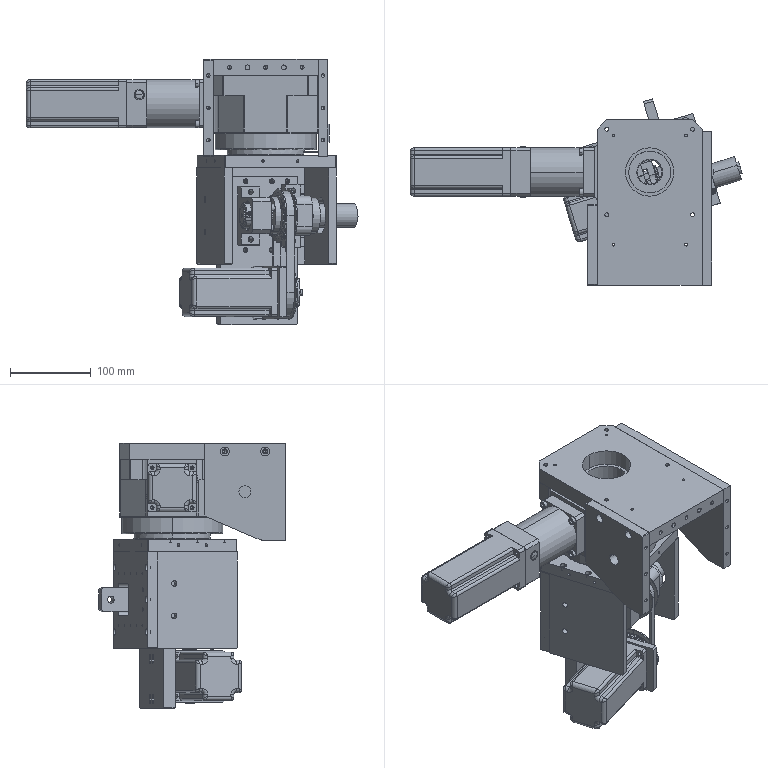Assembly | SolidWorks | mm | 53 component files | 55 solids | 3864 faces | box 411.09 x 231 x 328.5 mm | volume 4404841 mm3 | cylinder 1718 | plane 1389 | cone 489 | spline 222 | torus 46 | commonest cylinder face diameters 0.5 x176 0.4 x164 6.64 x156 5 x88 6 x86 52.53 x74 56.15 x72 3.3 x70
Bill of materials:
v1_Part1-2112091 | 1 |  | Thin-walled, closed band with an obround (stadium-shaped) outline: two straight parallel sides joined by semicircular ends, with a short constant axial width.
v1ZHXTbearingB6904ZZSB1 | 2 |  | Short annular body with a plain cylindrical bore, flat parallel faces, and concentric shallow recessed/stepped rings on the face. The overall look matches a sealed ball bearing.
V1ZHXTBearingMountingBaseSB1 | 1 |  | Block-style support with a large through-bore in a raised boss with chamfered corners, plus a thinner flange that sticks out on both sides and has one small through-hole in each tab. The overall look matches a shaft support or pillow-block bracket.
v1ZHXTRRING37SB1 | 1 |  | Thin flat split ring with two small lugs at the gap, each with a small round hole. The overall look matches a retaining ring (circlip).
V1ZHXTCylinderConnectionPlateSB1 | 1 |  | Rectangular block with chamfered corners, with one larger through-hole near one end and two smaller holes on an adjacent end face.
V1ZHXTGrindingBasePlateReinforcementPlateSB1 | 1 |  | Flat rectangular plate with two small through-holes near one edge on the main face and three small holes along one narrow edge face.
V1ZHXTGrindingBasePlateReinforcementRibSB1 | 1 |  | Flat rectangular plate with one large circular through-hole set off-center and three small holes along one narrow edge face.
v1ZHXTHG-KR23BSB1 | 1 |  | Simplified elongated rectangular housing with rounded edges and longitudinal recessed grooves on its sides. One end has a square flange with four corner holes, a circular pilot boss, and a protruding cylindrical shaft. The overall look matches a motor.
v1ZHXTHG-KR23SB1 | 1 |  | Elongated rectangular housing with rounded edges, longitudinal grooves, and a stepped/raised section at the rear end. The front has a square flange with four corner holes, a circular pilot, and a cylindrical shaft. The overall look matches a motor body.
v1ZHXTMGN12H--11SB1 | 2 |  | Long straight rail with a roughly rectangular cross-section, with longitudinal grooves along both sides near the top and a row of evenly spaced counterbored through-holes along its length. The overall look matches a linear guide rail.
v1ZHXTMGN12H-2SB1 | 4 |  | Rectangular carriage block with a channel underneath, with grooves inside the channel matching a rail profile. The flat top face has four holes in a rectangular pattern, and there are end plates/caps on both ends. The overall look matches a linear guide carriage.
V1ZHXTMotorMountingPlateSB1 | 1 |  | L-shaped bracket made from two plates at right angles. One plate has a large central circular opening with four small holes around it in a square pattern. The other leg has two mounting holes. Corners are chamfered.
v1ZHXTNKXRZ20SB1 | 1 |  | Stepped cylindrical sleeve or bushing with a through bore. The outer diameter has steps, and the outside has circumferential grooves. One end has a larger-diameter collar.
v1ZHXTHeadless_pin_DIN_913_M5x8SB1 | 3 |  | Short solid cylinder with a hexagonal socket recess in one end face and a chamfered or conical other end. The overall form looks like a set screw.
v1ZHXTPLNY20xSB1 | 1 |  | Annular ring with several rectangular slots evenly spaced around its outer edge and radial through-holes in the outer wall. The overall form looks like a slotted round nut or locking ring.
v1ZHXT14SB1 | 1 |  | Flanged hub: a circular flange with a central bore and a cylindrical, slightly tapered sleeve with a lengthwise slit on one side. Hex-socket cap-screw-like cylinders pass through the flange, and the flange also has plain holes.
v1ZHXTPTLA36P5M100_E_14_bodySB1 | 1 |  | Toothed pulley-like wheel with straight axial teeth and a raised disc flange on each side. It has a central bore and four small holes on a circle around the bore.
v1ZHXT20SB1 | 1 |  | Flanged hub similar to unnamed part 1: a circular flange with a central bore and a slit cylindrical sleeve on one side. Screw-like cylinders pass through the flange, and the flange also has plain holes.
v1ZHXTPTLA36P5M100_E_20_bodySB1 | 1 |  | Flanged toothed pulley-like wheel with straight axial teeth between two disc flanges and a central bore. Four small holes around the bore are visible from one face only.
V1ZHXTRotatingAxisMountingBaseSB1 | 1 |  | Bracket or support block: a flat mounting flange with two holes, joined to a body with rounded ends that holds a large cylindrical through bore. The bore axis is parallel to the mounting face.
V1ZHXTRotatingAxisSB1 | 1 |  | Stepped cylindrical shaft: a long, smaller-diameter section, a short intermediate step and a larger-diameter end section. The large end face has a small center hole, several small holes on a circle, and a circular step or groove.
V1ZHXTRotatingBasePlateSB1 | 1 |  | Thick rectangular plate with a large rectangular through cutout with rounded corners. It has rows of small holes, larger holes near the edges, and long shallow grooves across one face. One edge has a stepped or rebated strip.
V1ZHXTRotatingPlatformAdapterPlateSB1 | 1 | 6061 Alloy | Rectangular plate with a large central round through hole and many smaller holes in several sizes. The side edges also have holes.
V1ZHXTRotatingPlatformFixingPlateSB1 | 1 | 6061-O (SS) | Thick rectangular plate with two chamfered corners at one end, a large off-center round through hole, small holes in the face, and evenly spaced holes in the edge faces.
V1ZHXTRotatingSlideRailFixingPlateSB1 | 1 |  | Thin rectangular plate with many through holes: repeated groups of small holes in a grid, two clusters each with a larger central hole surrounded by smaller holes, and two pairs of short parallel slots toward one end.
V1ZHXT1,RR60BodySB1 | 1 |  | Housing-like body: a square flange with chamfered corners and four corner holes and a large central through bore, on top of a stepped cylindrical base; a cylindrical arm sticks out sideways and ends in a rectangular block with a small side hole.
V1ZHXT3.60InductionPlateSB1 | 1 |  | L-shaped bent bracket of thin sheet: a long flat leg with a rounded end and two through holes, and a short upright leg with a narrower stepped tab at the top.
v1ZHXTEE-SX672SB1 | 1 |  | Block-style bracket: an upright rectangular body with a slot cut into its bottom, forming two legs, and a horizontal cross-bar on top that extends into two rounded-end lugs, each with a through hole.
v1ZHXTHexagon socket button head screws GB_GB_SOCKET_TYPE7 M3X8-N_1SB1 | 4 |  | Pin with a plain cylindrical shank and a domed (round) head; looks like a rivet or round-head pin.
v1ZHXTHexagon socket countersunk head screws GB_GB_FASTENER_SCREWS_HSCHS M3X8-N_1SB1 | 8 |  | Pin with a cylindrical shank, a chamfered free end, and a conical head with a short cylindrical rim at its base; countersunk-head style.
v1ZHXTHexagon socket head cap screws GB_GB_FASTENER_SCREWS_HSHCS M5X20-N_1SB1 | 4 |  | Fastener-like pin: a cylindrical head with a rounded outer edge on a long cylindrical shank with a slightly chamfered end; resembles a socket-head cap screw envelope.
V1ZHXTZ-AxisConnectionPlateReinforcementRibSB1 | 1 |  | Thick flat plate with a mostly rectangular outline and one corner cut at an angle; it has a central through hole, two smaller holes near the top edge, and three small holes drilled into one narrow edge.
V1ZHXTZ-AxisMountingPlateReinforcementPlateSB1 | 1 |  | Tapered flat plate, like a gusset or bracket: tall at one end, sloping down along a straight angled edge toward the other end, with four evenly spaced holes along the long top edge and three small holes in the narrow edge at the tall end.
Mates:
1. concentric | V1ZHXTRotatingBasePlateSB1-1 face at (208.586, -137.891, 407.739) dir (-0.2918, 0.9565, 0) r 1.25 | v1ZHXTMGN12HSB1-1/v1ZHXTMGN12H--11SB1-1 face at (214.714, -157.977, 407.739) dir (0.2918, -0.9565, 0) r 1.75
2. concentric | V1ZHXTRotatingBasePlateSB1-1 face at (184.674, -145.187, 407.739) dir (-0.2918, 0.9565, 0) r 1.25 | v1ZHXTMGN12HSB1-1/v1ZHXTMGN12H--11SB1-1 face at (190.803, -165.272, 407.739) dir (0.2918, -0.9565, 0) r 1.75
3. concentric | V1ZHXTRotatingBasePlateSB1-1 face at (208.586, -137.891, 342.739) dir (-0.2918, 0.9565, 0) r 1.25 | v1ZHXTMGN12HSB1-2/v1ZHXTMGN12H--11SB1-1 face at (214.714, -157.977, 342.739) dir (0.2918, -0.9565, 0) r 1.75
4. concentric | V1ZHXTRotatingBasePlateSB1-1 face at (184.674, -145.187, 342.739) dir (-0.2918, 0.9565, 0) r 1.25 | v1ZHXTMGN12HSB1-2/v1ZHXTMGN12H--11SB1-1 face at (190.803, -165.272, 342.739) dir (0.2918, -0.9565, 0) r 1.75
5. coincident | V1ZHXTRotatingBasePlateSB1-1 face at (164.556, -164.917, 375.239) dir (0.2918, -0.9565, 0) | v1ZHXTMGN12HSB1-1/v1ZHXTMGN12H--11SB1-1 face at (164.556, -164.917, 407.739) dir (-0.2918, 0.9565, 0)
6. coincident | V1ZHXTRotatingBasePlateSB1-1 face at (164.556, -164.917, 375.239) dir (0.2918, -0.9565, 0) | v1ZHXTMGN12HSB1-2/v1ZHXTMGN12H--11SB1-1 face at (164.556, -164.917, 342.739) dir (-0.2918, 0.9565, 0)
7. coincident | v1ZHXTMGN12HSB1-2/v1ZHXTMGN12H-2SB1-3 face at (159.423, -180.074, 329.239) dir (0.2918, -0.9565, 0) | V1ZHXTRotatingSlideRailFixingPlateSB1-1 face at (163.536, -178.819, 375.239) dir (-0.2918, 0.9565, 0)
8. concentric | v1ZHXTMGN12HSB1-2/v1ZHXTMGN12H-2SB1-2 face at (198.926, -168.022, 332.739) dir (-0.2918, 0.9565, 0) r 1.5 | V1ZHXTRotatingSlideRailFixingPlateSB1-1 face at (203.303, -182.369, 332.739) dir (0.2918, -0.9565, 0) r 1.75
9. concentric | v1ZHXTMGN12HSB1-2/v1ZHXTMGN12H-2SB1-2 face at (198.926, -168.022, 352.739) dir (-0.2918, 0.9565, 0) r 1.5 | V1ZHXTRotatingSlideRailFixingPlateSB1-1 face at (203.303, -182.369, 352.739) dir (0.2918, -0.9565, 0) r 1.75
10. coincident | V1ZHXTRotatingSlideRailFixingPlateSB1-1 face at (167.914, -193.166, 375.239) dir (0.2918, -0.9565, 0) | V1ZHXTRotatingAxisMountingBaseSB1-1 face at (215.737, -178.575, 375.239) dir (-0.2918, 0.9565, 0)
11. concentric | V1ZHXTRotatingAxisMountingBaseSB1-1 face at (208.281, -222.67, 375.239) dir (0.9565, 0.2918, 0) r 18.5 | v1ZHXTNKXRZ20SB1-1 face at (209.238, -222.378, 375.239) dir (0.9565, 0.2918, 0) r 10
12. coincident | V1ZHXTRotatingAxisMountingBaseSB1-1 face at (234.123, -238.832, 336.239) dir (0.9565, 0.2918, 0) | v1ZHXTNKXRZ20SB1-1 face at (232.555, -233.696, 382.588) dir (-0.9565, -0.2918, 0)
13. concentric | V1ZHXTRotatingAxisSB1-1 face at (228.367, -216.542, 375.239) dir (-0.9565, -0.2918, 0) r 10 | v1ZHXTNKXRZ20SB1-1 face at (209.238, -222.378, 375.239) dir (0.9565, 0.2918, 0) r 10
14. coincident | V1ZHXTRotatingAxisSB1-1 face at (228.367, -216.542, 375.239) dir (-0.9565, -0.2918, 0) | v1ZHXTNKXRZ20SB1-1 face at (231.734, -227.577, 380.048) dir (0.9565, 0.2918, 0)
15. coincident | V1ZHXTRotatingSlideRailFixingPlateSB1-1 face at (167.914, -193.166, 375.239) dir (0.2918, -0.9565, 0) | V1ZHXTMotorMountingPlateSB1-1 face at (170.783, -192.291, 312.739) dir (-0.2918, 0.9565, 0)
16. coincident | V1ZHXTRotatingBasePlateSB1-1 face at (230.106, -131.325, 315.239) dir (0.9565, 0.2918, 0) | V1ZHXTRotatingPlatformAdapterPlateSB1-1 face at (223.394, -109.326, 435.239) dir (0.9565, 0.2918, 0)
17. coincident | V1ZHXTRotatingBasePlateSB1-1 face at (164.556, -164.917, 375.239) dir (0.2918, -0.9565, 0) | V1ZHXTGrindingBasePlateReinforcementPlateSB1-3 face at (104.777, -183.156, 435.239) dir (-0.2918, 0.9565, 0)
18. coincident | V1ZHXTRotatingPlatformAdapterPlateSB1-1 face at (230.106, -131.325, 435.239) dir (-0.2918, 0.9565, 0) | V1ZHXTRotatingBasePlateSB1-1 face at (160.762, -152.482, 375.239) dir (-0.2918, 0.9565, 0)
19. concentric | V1ZHXTRotatingSlideRailFixingPlateSB1-1 face at (170.232, -176.777, 255.239) dir (0.2918, -0.9565, 0) r 2.6 | V1ZHXTMotorMountingPlateSB1-1 face at (174.609, -191.124, 255.239) dir (-0.2918, 0.9565, 0) r 2.1
20. coincident | V1ZHXTRotatingSlideRailFixingPlateSB1-1 face at (167.914, -193.166, 375.239) dir (0.2918, -0.9565, 0) | v1ZHXTBGMWB6904ZZ_40SB1-1/V1ZHXTBearingMountingBaseSB1-1 face at (142.089, -201.046, 411.739) dir (-0.2918, 0.9565, 0)
21. concentric | V1ZHXTRotatingSlideRailFixingPlateSB1-1 face at (206.172, -181.493, 344.239) dir (0.2918, -0.9565, 0) r 2.5 | V1ZHXTRotatingAxisMountingBaseSB1-1 face at (206.172, -181.493, 344.239) dir (0.2918, -0.9565, 0) r 3.25
22. concentric | V1ZHXTRotatingSlideRailFixingPlateSB1-1 face at (206.172, -181.493, 406.239) dir (0.2918, -0.9565, 0) r 2.5 | V1ZHXTRotatingAxisMountingBaseSB1-1 face at (206.172, -181.493, 406.239) dir (0.2918, -0.9565, 0) r 3.25
23. concentric | V1ZHXTRotatingAxisSB1-1 face at (228.367, -216.542, 375.239) dir (-0.9565, -0.2918, 0) r 10 | v1ZHXTBGMWB6904ZZ_40SB1-1/v1ZHXTbearingB6904ZZSB1-1 face at (166.196, -235.511, 375.239) dir (-0.9565, -0.2918, 0) r 10
24. concentric | V1ZHXTRotatingSlideRailFixingPlateSB1-1 face at (153.567, -197.544, 404.739) dir (0.2918, -0.9565, 0) r 2.5 | v1ZHXTBGMWB6904ZZ_40SB1-1/V1ZHXTBearingMountingBaseSB1-1 face at (157.944, -211.891, 404.739) dir (-0.2918, 0.9565, 0) r 3.25
25. parallel | V1ZHXTMotorMountingPlateSB1-1 face at (190.108, -228.215, 280.239) dir (0.9565, 0.2918, 0) | v1ZHXTBGMWB6904ZZ_40SB1-1/V1ZHXTBearingMountingBaseSB1-1 face at (176.718, -232.301, 375.239) dir (0.9565, 0.2918, 0)
26. coincident | V1ZHXTRotatingPlatformAdapterPlateSB1-1 face at (176.521, -204.132, 435.239) dir (0, 0, -1) | V1ZHXTRotatingBasePlateSB1-1 face at (230.106, -131.325, 435.239) dir (0, 0, 1)
27. concentric | v1ZHXTMGN12HSB1-2/v1ZHXTMGN12H-2SB1-3 face at (128.147, -189.617, 352.739) dir (-0.2918, 0.9565, 0) r 1.5 | V1ZHXTRotatingSlideRailFixingPlateSB1-1 face at (132.524, -203.964, 352.739) dir (0.2918, -0.9565, 0) r 1.75
28. coincident | V1ZHXTRotatingPlatformAdapterPlateSB1-1 face at (176.521, -204.132, 435.239) dir (0, 0, -1) | V1ZHXTGrindingBasePlateReinforcementRibSB1-1 face at (224.335, -146.677, 435.239) dir (0, 0, 1)
29. coincident | V1ZHXTRotatingBasePlateSB1-1 face at (164.556, -164.917, 375.239) dir (0.2918, -0.9565, 0) | V1ZHXTGrindingBasePlateReinforcementRibSB1-1 face at (224.335, -146.677, 435.239) dir (-0.2918, 0.9565, 0)
30. coincident | V1ZHXTRotatingBasePlateSB1-1 face at (230.106, -131.325, 315.239) dir (0.9565, 0.2918, 0) | V1ZHXTGrindingBasePlateReinforcementRibSB1-1 face at (248.929, -193.017, 375.239) dir (0.9565, 0.2918, 0)
31. coincident | V1ZHXTRotatingPlatformAdapterPlateSB1-1 face at (176.521, -204.132, 435.239) dir (0, 0, -1) | V1ZHXTGrindingBasePlateReinforcementPlateSB1-3 face at (104.777, -183.156, 435.239) dir (0, 0, 1)
32. coincident | V1ZHXTRotatingPlatformAdapterPlateSB1-1 face at (84.706, -151.641, 435.239) dir (-0.9565, -0.2918, 0) | V1ZHXTGrindingBasePlateReinforcementPlateSB1-3 face at (110.241, -235.332, 375.239) dir (-0.9565, -0.2918, 0)
33. coincident | V1ZHXTRotatingPlatformAdapterPlateSB1-1 face at (176.521, -204.132, 450.239) dir (0, 0, 1) | V1ZHXTRR60SecondarySB1-1/V1ZHXT1,RR60BodySB1-1 face at (176.521, -204.132, 450.239) dir (0, 0, -1)
34. concentric | v1ZHXTHG-KR23BSB1-1 face at (34.521, -204.132, 513.739) dir (-1, 0, 0) r 7 | V1ZHXTRR60SecondarySB1-1/V1ZHXT1,RR60BodySB1-1 face at (36.521, -204.132, 513.739) dir (-1, 0, 0) r 7
35. coincident | v1ZHXTHG-KR23BSB1-1 face at (4.521, -204.132, 513.739) dir (1, 0, 0) | V1ZHXTRR60SecondarySB1-1/V1ZHXT1,RR60BodySB1-1 face at (4.521, -174.132, 543.739) dir (-1, 0, 0)
36. coincident | v1ZHXTHG-KR23BSB1-1 face at (-120.279, -174.132, 543.739) dir (0, 1, 0) | V1ZHXTRR60SecondarySB1-1/V1ZHXT1,RR60BodySB1-1 face at (4.521, -174.132, 543.739) dir (0, 1, 0)
37. coincident | V1ZHXTRotatingPlatformFixingPlateSB1-1 face at (176.521, -204.132, 548.739) dir (0, 0, -1) | V1ZHXTRR60SecondarySB1-1/V1ZHXT1,RR60BodySB1-1 face at (241.521, -139.132, 548.739) dir (0, 0, 1)
38. concentric | V1ZHXTRotatingPlatformFixingPlateSB1-1 face at (123.488, -151.099, 548.739) dir (0, 0, -1) r 2.5 | V1ZHXTRR60SecondarySB1-1/V1ZHXT1,RR60BodySB1-1 face at (123.488, -151.099, 523.739) dir (0, 0, -1) r 3.3
39. concentric | V1ZHXTRotatingPlatformFixingPlateSB1-1 face at (123.488, -257.165, 548.739) dir (0, 0, -1) r 2.5 | V1ZHXTRR60SecondarySB1-1/V1ZHXT1,RR60BodySB1-1 face at (123.488, -257.165, 523.739) dir (0, 0, -1) r 3.3
40. concentric | V1ZHXTRotatingPlatformAdapterPlateSB1-1 face at (176.521, -204.132, 450.239) dir (0, 0, -1) r 16 | V1ZHXTRR60SecondarySB1-1/V1ZHXT1,RR60BodySB1-1 face at (176.521, -204.132, 548.739) dir (0, 0, -1) r 15
41. concentric | V1ZHXTZ-AxisMountingPlateReinforcementPlateSB1-1 face at (253.521, -319.132, 558.739) dir (1, 0, 0) r 3.2 | V1ZHXTRotatingPlatformFixingPlateSB1-1 face at (241.521, -319.132, 558.739) dir (1, 0, 0) r 2.5
42. coincident | V1ZHXTZ-AxisMountingPlateReinforcementPlateSB1-1 face at (241.521, -249.132, 508.739) dir (-1, 0, 0) | V1ZHXTRotatingPlatformFixingPlateSB1-1 face at (241.521, -64.132, 548.739) dir (1, 0, 0)
43. coincident | V1ZHXTMotorMountingPlateSB1-1 face at (182.456, -230.55, 280.239) dir (-0.9565, -0.2918, 0) | v1ZHXTHG-KR23SB1-1 face at (182.456, -230.55, 280.239) dir (0.9565, 0.2918, 0)
44. concentric | V1ZHXTMotorMountingPlateSB1-1 face at (189.679, -254.221, 255.49) dir (-0.9565, -0.2918, 0) r 1.65 | v1ZHXTHG-KR23SB1-1 face at (84.754, -286.235, 255.49) dir (0.9565, 0.2918, 0) r 2.25
45. concentric | V1ZHXTMotorMountingPlateSB1-1 face at (190.108, -228.215, 280.239) dir (-0.9565, -0.2918, 0) r 25 | v1ZHXTHG-KR23SB1-1 face at (185.326, -229.674, 280.239) dir (-0.9565, -0.2918, 0) r 25
46. concentric | v1ZHXTHG-KR23SB1-1 face at (211.15, -221.795, 280.239) dir (-0.9565, -0.2918, 0) r 7 | v1ZHXTPTLA36P5M100_E_14SB1-1/v1ZHXT14SB1-1 face at (192.978, -227.34, 280.239) dir (0.9565, 0.2918, 0) r 7
47. distance | v1ZHXTPTLA36P5M100_E_14SB1-1/v1ZHXTPTLA36P5M100_E_14_bodySB1-1 face at (189.022, -221.228, 280.239) dir (-0.9565, -0.2918, 0) | V1ZHXTMotorMountingPlateSB1-1 face at (190.108, -228.215, 280.239) dir (0.9565, 0.2918, 0)
48. concentric | V1ZHXTRotatingAxisSB1-1 face at (228.367, -216.542, 375.239) dir (-0.9565, -0.2918, 0) r 10 | v1ZHXTPTLA36P5M100_E_20SB1-1/v1ZHXT20SB1-1 face at (204.455, -223.838, 375.239) dir (-0.9565, -0.2918, 0) r 10
49. distance | v1ZHXTPTLA36P5M100_E_20SB1-1/v1ZHXTPTLA36P5M100_E_20_bodySB1-1 face at (203.908, -215.192, 369.858) dir (0.9565, 0.2918, 0) | V1ZHXTRotatingAxisMountingBaseSB1-1 face at (214.993, -244.669, 336.239) dir (-0.9565, -0.2918, 0)
50. coincident | V1ZHXTRotatingSlideRailFixingPlateSB1-1 face at (163.536, -178.819, 375.239) dir (-0.2918, 0.9565, 0) | V1ZHXTCylinderConnectionPlateSB1-1 face at (191.274, -170.356, 375.239) dir (0.2918, -0.9565, 0)
51. concentric | V1ZHXTRotatingSlideRailFixingPlateSB1-1 face at (195.651, -184.703, 383.239) dir (0.2918, -0.9565, 0) r 2.65 | V1ZHXTCylinderConnectionPlateSB1-1 face at (191.274, -170.356, 383.239) dir (0.2918, -0.9565, 0) r 2.1
52. coincident | V1ZHXTRotatingPlatformFixingPlateSB1-1 face at (111.521, -64.132, 548.739) dir (-1, 0, 0) | V1ZHXTZ-AxisConnectionPlateReinforcementRibSB1-1 face at (111.521, -294.132, 508.739) dir (1, 0, 0)
53. coincident | V1ZHXTRotatingPlatformFixingPlateSB1-1 face at (176.521, -204.132, 568.739) dir (0, 0, 1) | V1ZHXTZ-AxisConnectionPlateReinforcementRibSB1-1 face at (111.521, -244.132, 568.739) dir (0, 0, 1)
54. concentric | v1ZHXTMGN12HSB1-1/v1ZHXTMGN12H-2SB1-3 face at (128.147, -189.617, 417.739) dir (-0.2918, 0.9565, 0) r 1.5 | V1ZHXTRotatingSlideRailFixingPlateSB1-1 face at (132.524, -203.964, 417.739) dir (0.2918, -0.9565, 0) r 1.75
55. concentric | v1ZHXTMGN12HSB1-1/v1ZHXTMGN12H-2SB1-2 face at (198.926, -168.022, 417.739) dir (-0.2918, 0.9565, 0) r 1.5 | V1ZHXTRotatingSlideRailFixingPlateSB1-1 face at (203.303, -182.369, 417.739) dir (0.2918, -0.9565, 0) r 1.75
56. concentric | V1ZHXTRotatingAxisSB1-1 face at (228.367, -216.542, 375.239) dir (-0.9565, -0.2918, 0) r 10 | v1ZHXTPLNY20SB1-1/v1ZHXTPLNY20xSB1-1 face at (148.023, -241.056, 375.239) dir (0.9565, 0.2918, 0) r 10.01
57. coincident | v1ZHXTBGMWB6904ZZ_40SB1-1/v1ZHXTbearingB6904ZZSB1-1 face at (153.882, -225.99, 375.239) dir (-0.9565, -0.2918, 0) | v1ZHXTPLNY20SB1-1/v1ZHXTPLNY20xSB1-1 face at (157.588, -238.137, 375.239) dir (0.9565, 0.2918, 0)
58. concentric | V1ZHXTRotatingPlatformFixingPlateSB1-1 face at (111.521, -319.132, 558.739) dir (-1, 0, 0) r 2.5 | V1ZHXTZ-AxisConnectionPlateReinforcementRibSB1-1 face at (99.521, -319.132, 558.739) dir (-1, 0, 0) r 3.2
59. parallel | V1ZHXTZ-AxisMountingPlateReinforcementPlateSB1-1 face at (253.521, -154.132, 568.739) dir (0, 0, 1) | V1ZHXTRotatingPlatformFixingPlateSB1-1 face at (176.521, -204.132, 568.739) dir (0, 0, 1)
60. concentric | v1ZHXTPTLA36P5M100_E_14SB1-1/v1ZHXT14SB1-1 face at (192.978, -227.34, 280.239) dir (0.9565, 0.2918, 0) r 17.5 | v1_Part1-2112091-1 face at (203.499, -224.129, 280.239) dir (-0.9565, -0.2918, 0) r 30.1
61. width | v1ZHXTPTLA36P5M100_E_14SB1-1/v1ZHXTPTLA36P5M100_E_14_bodySB1-1 face at (184.808, -199.878, 280.239) dir (0.9565, 0.2918, 0) | v1ZHXTPTLA36P5M100_E_14SB1-1/v1ZHXTPTLA36P5M100_E_14_bodySB1-1 face at (196.071, -197.043, 280.239) dir (-0.9565, -0.2918, 0) | v1_Part1-2112091-1 face at (203.499, -224.129, 280.239) dir (0.9565, 0.2918, 0) | v1_Part1-2112091-1 face at (193.934, -227.048, 280.239) dir (-0.9565, -0.2918, 0)
62. concentric | v1ZHXTPTLA36P5M100_E_20SB1-1/v1ZHXT20SB1-1 face at (204.455, -223.838, 375.239) dir (-0.9565, -0.2918, 0) r 23 | v1_Part1-2112091-1 face at (203.499, -224.129, 375.239) dir (-0.9565, -0.2918, 0) r 28.1
63. distance | v1ZHXTbearingB6904ZZSB1-1 plane at (0, 0, 8) dir (0, 0, -1) | V1ZHXTBearingMountingBaseSB1-1 plane at (0, 0, 8) dir (0, 0, 1)
64. coincident | V1ZHXTBearingMountingBaseSB1-1 axis at (0, 0, 80.9) dir (0, 0, -1) | v1ZHXTbearingB6904ZZSB1-1 axis at (0, 0, -72.9) dir (0, 0, 1)
65. coincident | V1ZHXTBearingMountingBaseSB1-1 axis at (0, 0, 80.9) dir (0, 0, -1) | v1ZHXTbearingB6904ZZSB1-1 axis at (0, 0, -72.9) dir (0, 0, 1)
66. coincident | V1ZHXTBearingMountingBaseSB1-1 axis at (0, 0, 80.9) dir (0, 0, -1) | v1ZHXTbearingB6904ZZSB1-1 axis at (0, 0, -72.9) dir (0, 0, 1)
67. angle | v1ZHXTbearingB6904ZZSB1-1 plane at (0, 0, 8) dir (1, 0, 0) | V1ZHXTBearingMountingBaseSB1-1 plane at (0, 0, 0) dir (1, 0, 0)
68. distance | v1ZHXTRRING37SB1-1 plane at (0, 0, 9.6) dir (0, 0, -1) | V1ZHXTBearingMountingBaseSB1-1 plane at (0, 0, 9.6) dir (0, 0, 1)
69. coincident | V1ZHXTBearingMountingBaseSB1-1 axis at (0, 0, 80.9) dir (0, 0, -1) | v1ZHXTRRING37SB1-1 axis at (0, 0, -71.3) dir (0, 0, 1)
70. coincident | V1ZHXTBearingMountingBaseSB1-1 axis at (0, 0, 80.9) dir (0, 0, -1) | v1ZHXTRRING37SB1-1 axis at (0, 0, -71.3) dir (0, 0, 1)
71. angle | v1ZHXTRRING37SB1-1 plane at (0, 0, 9.6) dir (0, -1, 0) | V1ZHXTBearingMountingBaseSB1-1 plane at (0, 0, 0) dir (1, 0, 0)
72. distance | v1ZHXTbearingB6904ZZSB1-2 sketch point at (0, 0, -10) dir (1, 0, 0) | V1ZHXTBearingMountingBaseSB1-1 plane at (0, 0, -10) dir (0, 0, 1)
73. coincident | V1ZHXTBearingMountingBaseSB1-1 axis at (0, 0, 80.9) dir (0, 0, -1) | v1ZHXTbearingB6904ZZSB1-2 sketch point at (0, 0, -10) dir (1, 0, 0)
74. angle | V1ZHXTBearingMountingBaseSB1-1 axis at (-80.9, 0, -10) dir (1, 0, 0) | v1ZHXTbearingB6904ZZSB1-2 axis at (-80.9, 0, -10) dir (1, 0, 0)
75. angle | V1ZHXTBearingMountingBaseSB1-1 axis at (0, 0, 80.9) dir (0, 0, -1) | v1ZHXTbearingB6904ZZSB1-2 axis at (0, 0, 70.9) dir (0, 0, -1)
76. coincident | v1ZHXTMGN12H--11SB1-1 face at (104.48, 63.892, 2.939) dir (0, 1, 0) | v1ZHXTMGN12H-2SB1-2 face at (110.48, 63.892, 71.157) dir (0, -1, 0)
77. width | v1ZHXTMGN12H-2SB1-2 face at (98.48, 60.142, 71.157) dir (1, 0, 0) | v1ZHXTMGN12H-2SB1-2 face at (110.48, 55.892, 71.157) dir (-1, 0, 0) | v1ZHXTMGN12H--11SB1-1 face at (98.48, 63.892, 62.939) dir (-1, 0, 0) | v1ZHXTMGN12H--11SB1-1 face at (110.48, 63.892, -57.061) dir (1, 0, 0)
78. coincident | v1ZHXTMGN12H--11SB1-1 face at (104.48, 63.892, 2.939) dir (0, 1, 0) | v1ZHXTMGN12H-2SB1-3 face at (110.48, 63.892, 17.377) dir (0, -1, 0)
79. width | v1ZHXTMGN12H-2SB1-3 face at (110.48, 55.892, 17.377) dir (-1, 0, 0) | v1ZHXTMGN12H-2SB1-3 face at (98.48, 60.142, 17.377) dir (1, 0, 0) | v1ZHXTMGN12H--11SB1-1 face at (110.48, 63.892, -57.061) dir (1, 0, 0) | v1ZHXTMGN12H--11SB1-1 face at (98.48, 63.892, 62.939) dir (-1, 0, 0)
80. distance | v1ZHXTHeadless_pin_DIN_913_M5x8SB1-1 plane at (5.5, 16.2, 0) dir (0, -1, 0) | v1ZHXTPLNY20xSB1-1 plane at (0, 16.2, 0) dir (0, 1, 0)
81. coincident | v1ZHXTPLNY20xSB1-1 axis at (5.5, 50, 0) dir (0, -1, 0) | v1ZHXTHeadless_pin_DIN_913_M5x8SB1-1 axis at (5.5, -64.7, 0) dir (0, 1, 0)
82. coincident | v1ZHXTPLNY20xSB1-1 axis at (5.5, 50, 0) dir (0, -1, 0) | v1ZHXTHeadless_pin_DIN_913_M5x8SB1-1 axis at (5.5, -64.7, 0) dir (0, 1, 0)
83. coincident | v1ZHXTPLNY20xSB1-1 axis at (5.5, 50, 0) dir (0, -1, 0) | v1ZHXTHeadless_pin_DIN_913_M5x8SB1-1 axis at (5.5, -64.7, 0) dir (0, 1, 0)
84. angle | v1ZHXTHeadless_pin_DIN_913_M5x8SB1-1 plane at (5.5, 16.2, 0) dir (1, 0, 0) | v1ZHXTPLNY20xSB1-1 plane at (5.5, 0, 0) dir (1, 0, 0)
85. distance | v1ZHXTHeadless_pin_DIN_913_M5x8SB1-2 plane at (5.5, -5.541, -15.223) dir (0, 0.342, 0.9397) | v1ZHXTPLNY20xSB1-1 plane at (0, -5.541, -15.223) dir (0, -0.342, -0.9397)
86. coincident | v1ZHXTPLNY20xSB1-1 axis at (5.5, -29.445, -80.9) dir (0, 0.342, 0.9397) | v1ZHXTHeadless_pin_DIN_913_M5x8SB1-2 axis at (5.5, 22.129, 60.798) dir (0, -0.342, -0.9397)
87. coincident | v1ZHXTPLNY20xSB1-1 axis at (5.5, -29.445, -80.9) dir (0, 0.342, 0.9397) | v1ZHXTHeadless_pin_DIN_913_M5x8SB1-2 axis at (5.5, 22.129, 60.798) dir (0, -0.342, -0.9397)
88. coincident | v1ZHXTPLNY20xSB1-1 axis at (5.5, -29.445, -80.9) dir (0, 0.342, 0.9397) | v1ZHXTHeadless_pin_DIN_913_M5x8SB1-2 axis at (5.5, 22.129, 60.798) dir (0, -0.342, -0.9397)
89. angle | v1ZHXTHeadless_pin_DIN_913_M5x8SB1-2 plane at (5.5, -5.541, -15.223) dir (1, 0, 0) | v1ZHXTPLNY20xSB1-1 plane at (5.5, 0, 0) dir (1, 0, 0)
90. distance | v1ZHXTHeadless_pin_DIN_913_M5x8SB1-3 plane at (5.5, -5.541, 15.223) dir (0, 0.342, -0.9397) | v1ZHXTPLNY20xSB1-1 plane at (0, -5.541, 15.223) dir (0, -0.342, 0.9397)
91. coincident | v1ZHXTPLNY20xSB1-1 axis at (5.5, -29.445, 80.9) dir (0, 0.342, -0.9397) | v1ZHXTHeadless_pin_DIN_913_M5x8SB1-3 axis at (5.5, 22.129, -60.798) dir (0, -0.342, 0.9397)
92. coincident | v1ZHXTPLNY20xSB1-1 axis at (5.5, -29.445, 80.9) dir (0, 0.342, -0.9397) | v1ZHXTHeadless_pin_DIN_913_M5x8SB1-3 axis at (5.5, 22.129, -60.798) dir (0, -0.342, 0.9397)
93. coincident | v1ZHXTPLNY20xSB1-1 axis at (5.5, -29.445, 80.9) dir (0, 0.342, -0.9397) | v1ZHXTHeadless_pin_DIN_913_M5x8SB1-3 axis at (5.5, 22.129, -60.798) dir (0, -0.342, 0.9397)
94. angle | v1ZHXTHeadless_pin_DIN_913_M5x8SB1-3 plane at (5.5, -5.541, 15.223) dir (1, 0, 0) | v1ZHXTPLNY20xSB1-1 plane at (5.5, 0, 0) dir (1, 0, 0)
95. distance | v1ZHXT14SB1-1 plane at (-12, 0, 0) dir (1, 0, 0) | v1ZHXTPTLA36P5M100_E_14_bodySB1-1 plane at (-12, 0, 0) dir (1, 0, 0)
96. coincident | v1ZHXTPTLA36P5M100_E_14_bodySB1-1 axis at (80.9, 0, 0) dir (-1, 0, 0) | v1ZHXT14SB1-1 axis at (72.9, 0, 0) dir (-1, 0, 0)
97. coincident | v1ZHXTPTLA36P5M100_E_14_bodySB1-1 axis at (80.9, 0, 0) dir (-1, 0, 0) | v1ZHXT14SB1-1 axis at (72.9, 0, 0) dir (-1, 0, 0)
98. coincident | v1ZHXTPTLA36P5M100_E_14_bodySB1-1 axis at (80.9, 0, 0) dir (-1, 0, 0) | v1ZHXT14SB1-1 axis at (72.9, 0, 0) dir (-1, 0, 0)
99. angle | v1ZHXT14SB1-1 plane at (-8, 0, 0) dir (0, 0, -1) | v1ZHXTPTLA36P5M100_E_14_bodySB1-1 plane at (0, 0, 0) dir (0, 0, -1)
100. distance | v1ZHXT20SB1-1 plane at (-14, 0, 0) dir (1, 0, 0) | v1ZHXTPTLA36P5M100_E_20_bodySB1-1 plane at (-14, 0, 0) dir (1, 0, 0)
101. coincident | v1ZHXTPTLA36P5M100_E_20_bodySB1-1 axis at (80.9, 0, 0) dir (-1, 0, 0) | v1ZHXT20SB1-1 axis at (71.9, 0, 0) dir (-1, 0, 0)
102. coincident | v1ZHXTPTLA36P5M100_E_20_bodySB1-1 axis at (80.9, 0, 0) dir (-1, 0, 0) | v1ZHXT20SB1-1 axis at (71.9, 0, 0) dir (-1, 0, 0)
103. coincident | v1ZHXTPTLA36P5M100_E_20_bodySB1-1 axis at (80.9, 0, 0) dir (-1, 0, 0) | v1ZHXT20SB1-1 axis at (71.9, 0, 0) dir (-1, 0, 0)
104. angle | v1ZHXT20SB1-1 plane at (-9, 0, 0) dir (0, 0, -1) | v1ZHXTPTLA36P5M100_E_20_bodySB1-1 plane at (0, 0, 0) dir (0, 0, -1)